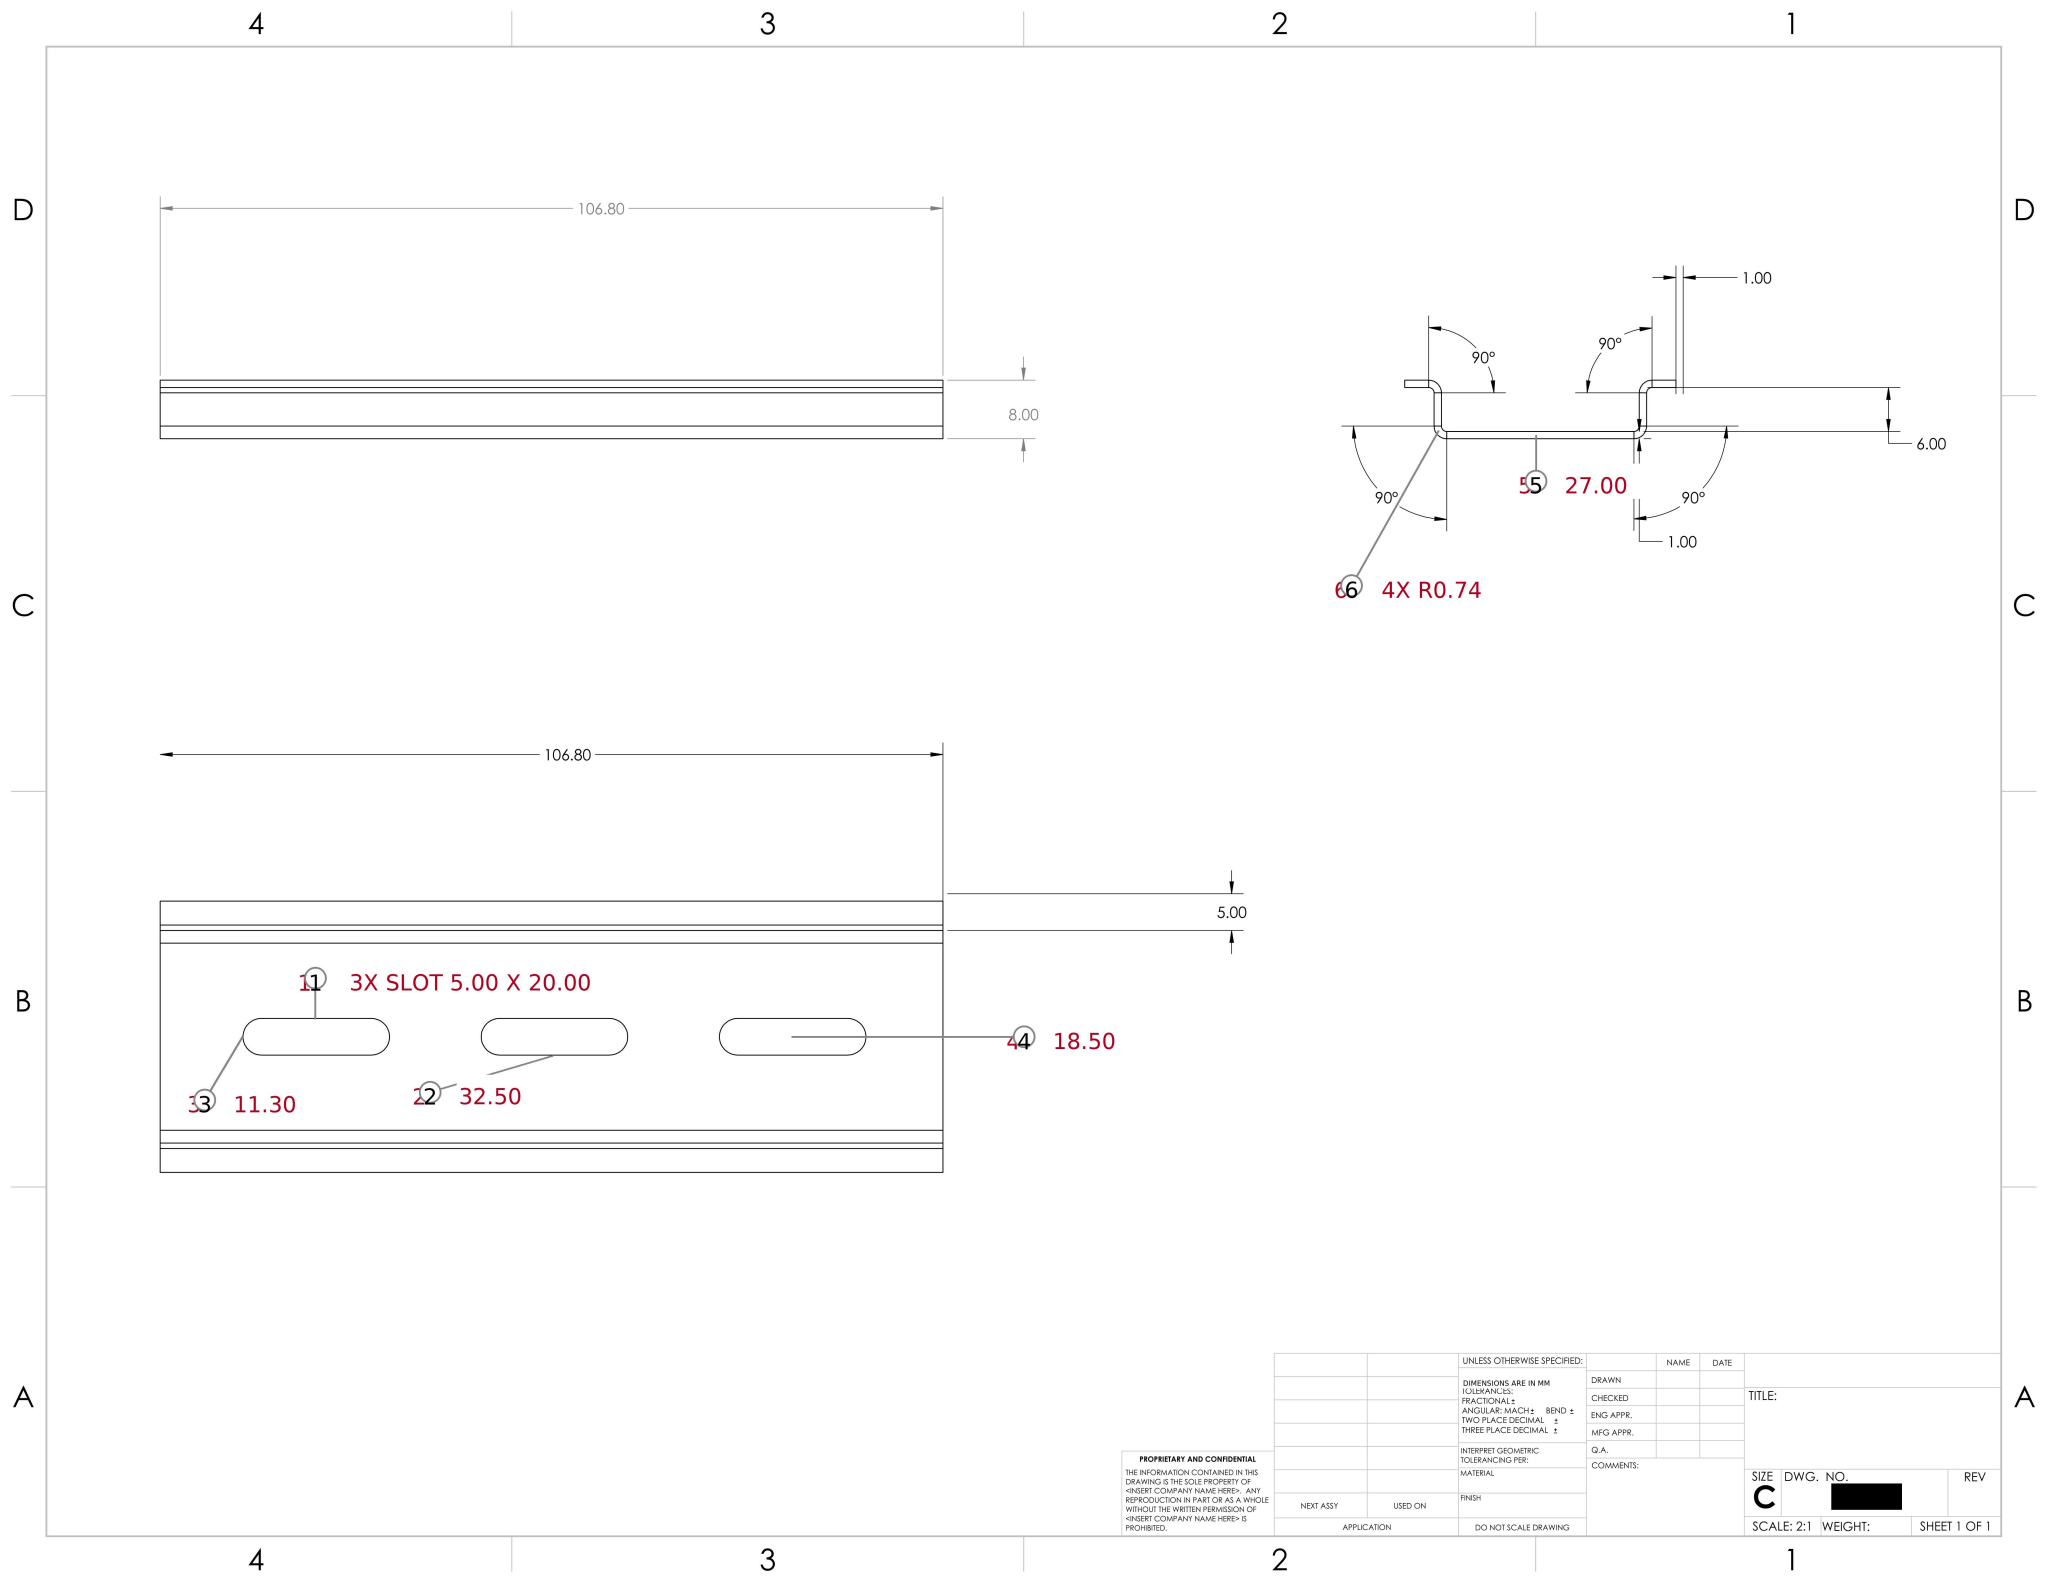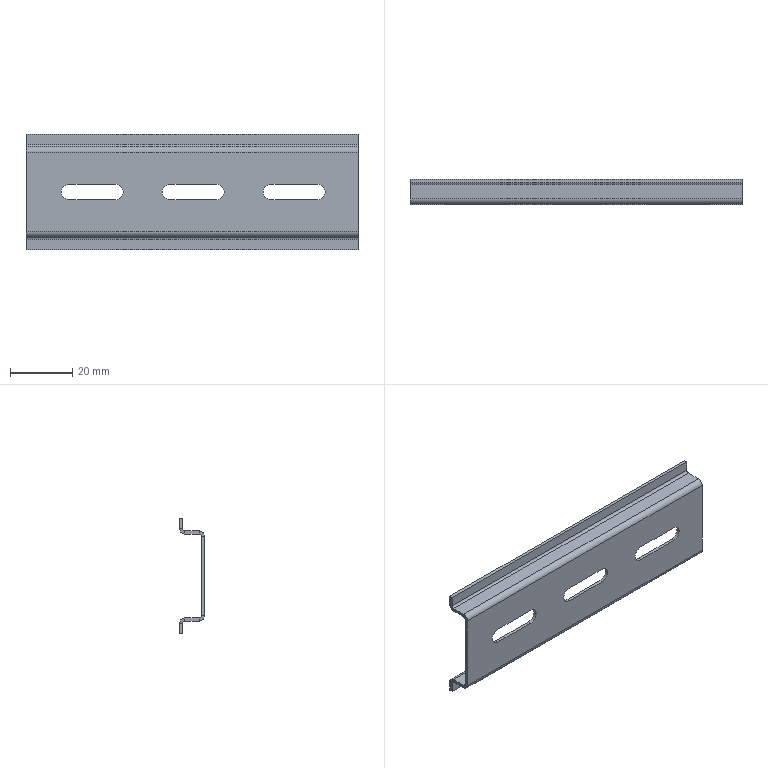Part | SolidWorks | mm | 1 solid | 50 faces | box 106.8 x 8 x 37 mm | volume 4936 mm3 | plane 36 | cylinder 14 | commonest cylinder face diameters 5 x6 3.473 x4 1.473 x4